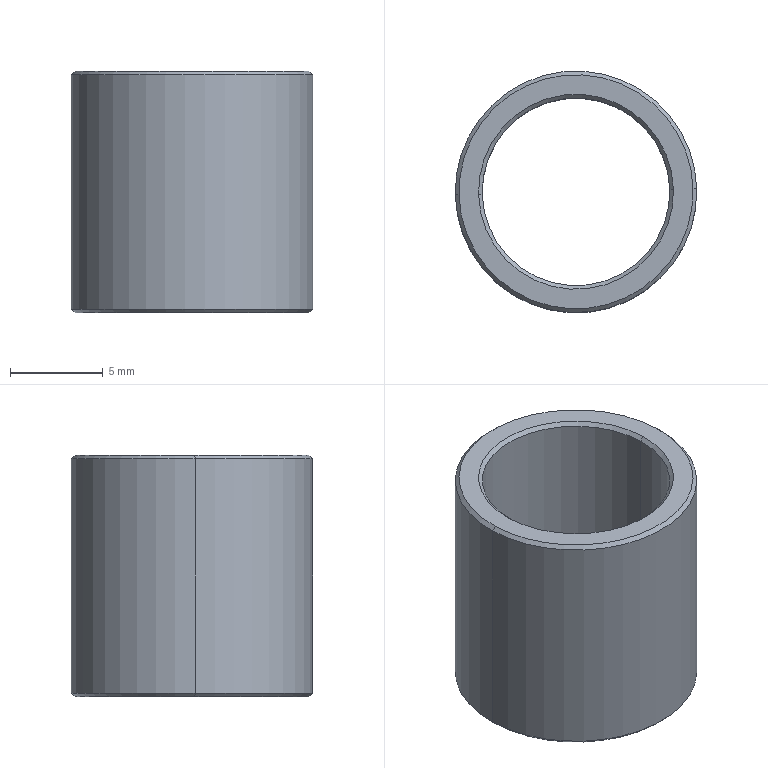Component | SolidWorks | 170423A4-IdlerAssembly5-10_170423A4-AxisCollar-1 | 1 solid | 14 faces | box 13 x 13 x 13 mm | volume 681 mm3 | cone 8 | cylinder 4 | plane 2 | commonest cylinder face diameters 10.1 x2 13 x2
build123d program:
from build123d import *

# Parameters (mm, degrees)
SKETCH1_R           = 6.5
SKETCH1_R_2         = 5.05
BOSS_EXTRUDE1_DEPTH = 13
CHAMFER1_SIZE       = 0.2


with BuildPart() as part:
    # Sketch1 → Boss-Extrude1 (new body)
    with BuildSketch(Plane.XY):
        with Locations(Location((0, 0, 0), (0, 0, 180))):
            Circle(SKETCH1_R)
        with Locations(Location((0, 0, 0), (0, 0, 180))):
            Circle(SKETCH1_R_2, mode=Mode.SUBTRACT)
    extrude(amount=BOSS_EXTRUDE1_DEPTH)

    # Chamfer1
    chamfer1_edges = [part.edges().sort_by_distance(p)[0] for p in [
        (6.5, 0, 0),
        (6.5, 0, 13),
        (5.05, 0, 0),
        (5.05, 0, 13),
    ]]
    chamfer(chamfer1_edges, length=CHAMFER1_SIZE)


solid = part.part

# Placed as in the assembly
solid = solid.moved(Location((-162.746, 8.712, 437.5), (0, 0, 0)))
STEP:
#1=COLOUR_RGB('',0.7922,0.8196,0.9333);
#2=FILL_AREA_STYLE_COLOUR('',#1);
#3=FILL_AREA_STYLE('',(#2));
#4=SURFACE_STYLE_FILL_AREA(#3);
#5=SURFACE_SIDE_STYLE('',(#4));
#6=SURFACE_STYLE_USAGE(.BOTH.,#5);
#7=PRESENTATION_STYLE_ASSIGNMENT((#6));
#8=CARTESIAN_POINT('',(-6.209,0.348,17.728));
#9=VERTEX_POINT('',#8);
#10=CARTESIAN_POINT('',(-6.606,0.3379,17.728));
#11=VERTEX_POINT('',#10);
#12=CARTESIAN_POINT('',(-6.407,0.343,17.728));
#13=DIRECTION('',(0.,0.,1.));
#14=DIRECTION('',(-0.9997,-0.02534,0.));
#15=AXIS2_PLACEMENT_3D('',#12,#13,#14);
#16=CIRCLE('',#15,0.1988);
#17=EDGE_CURVE('',#9,#11,#16,.T.);
#18=ORIENTED_EDGE('',*,*,#17,.F.);
#19=CARTESIAN_POINT('',(-6.201,0.3482,17.736));
#20=VERTEX_POINT('',#19);
#21=CARTESIAN_POINT('',(-6.209,0.348,17.728));
#22=DIRECTION('',(0.7069,0.01792,0.7071));
#23=VECTOR('',#22,39.37);
#24=LINE('',#21,#23);
#25=EDGE_CURVE('',#9,#20,#24,.T.);
#26=ORIENTED_EDGE('',*,*,#25,.T.);
#27=CARTESIAN_POINT('',(-6.614,0.3377,17.736));
#28=VERTEX_POINT('',#27);
#29=CARTESIAN_POINT('',(-6.407,0.343,17.736));
#30=DIRECTION('',(0.,0.,-1.));
#31=DIRECTION('',(-0.9997,-0.02534,0.));
#32=AXIS2_PLACEMENT_3D('',#29,#30,#31);
#33=CIRCLE('',#32,0.2067);
#34=EDGE_CURVE('',#28,#20,#33,.T.);
#35=ORIENTED_EDGE('',*,*,#34,.F.);
#36=CARTESIAN_POINT('',(-6.606,0.3379,17.728));
#37=DIRECTION('',(-0.7069,-0.01792,0.7071));
#38=VECTOR('',#37,39.37);
#39=LINE('',#36,#38);
#40=EDGE_CURVE('',#11,#28,#39,.T.);
#41=ORIENTED_EDGE('',*,*,#40,.F.);
#42=EDGE_LOOP('',(#18,#26,#35,#41));
#43=FACE_OUTER_BOUND('',#42,.T.);
#44=CARTESIAN_POINT('',(-6.407,0.343,17.728));
#45=DIRECTION('',(0.,0.,1.));
#46=DIRECTION('',(-0.9997,-0.02534,0.));
#47=AXIS2_PLACEMENT_3D('',#44,#45,#46);
#48=CONICAL_SURFACE('',#47,0.1988,0.7854);
#49=ADVANCED_FACE('',(#43),#48,.F.);
#50=CARTESIAN_POINT('',(-6.655,0.3367,17.736));
#51=VERTEX_POINT('',#50);
#52=CARTESIAN_POINT('',(-6.159,0.3493,17.736));
#53=VERTEX_POINT('',#52);
#54=CARTESIAN_POINT('',(-6.407,0.343,17.736));
#55=DIRECTION('',(0.,0.,1.));
#56=DIRECTION('',(-0.9997,-0.02534,0.));
#57=AXIS2_PLACEMENT_3D('',#54,#55,#56);
#58=CIRCLE('',#57,0.248);
#59=EDGE_CURVE('',#51,#53,#58,.T.);
#60=ORIENTED_EDGE('',*,*,#59,.F.);
#61=CARTESIAN_POINT('',(-6.663,0.3365,17.728));
#62=VERTEX_POINT('',#61);
#63=CARTESIAN_POINT('',(-6.655,0.3367,17.736));
#64=DIRECTION('',(-0.7069,-0.01792,-0.7071));
#65=VECTOR('',#64,39.37);
#66=LINE('',#63,#65);
#67=EDGE_CURVE('',#51,#62,#66,.T.);
#68=ORIENTED_EDGE('',*,*,#67,.T.);
#69=CARTESIAN_POINT('',(-6.152,0.3495,17.728));
#70=VERTEX_POINT('',#69);
#71=CARTESIAN_POINT('',(-6.407,0.343,17.728));
#72=DIRECTION('',(0.,0.,-1.));
#73=DIRECTION('',(-0.9997,-0.02534,0.));
#74=AXIS2_PLACEMENT_3D('',#71,#72,#73);
#75=CIRCLE('',#74,0.2559);
#76=EDGE_CURVE('',#70,#62,#75,.T.);
#77=ORIENTED_EDGE('',*,*,#76,.F.);
#78=CARTESIAN_POINT('',(-6.159,0.3493,17.736));
#79=DIRECTION('',(0.7069,0.01792,-0.7071));
#80=VECTOR('',#79,39.37);
#81=LINE('',#78,#80);
#82=EDGE_CURVE('',#53,#70,#81,.T.);
#83=ORIENTED_EDGE('',*,*,#82,.F.);
#84=EDGE_LOOP('',(#60,#68,#77,#83));
#85=FACE_OUTER_BOUND('',#84,.T.);
#86=CARTESIAN_POINT('',(-6.407,0.343,17.736));
#87=DIRECTION('',(0.,0.,-1.));
#88=DIRECTION('',(0.9997,0.02534,0.));
#89=AXIS2_PLACEMENT_3D('',#86,#87,#88);
#90=CONICAL_SURFACE('',#89,0.248,0.7854);
#91=ADVANCED_FACE('',(#85),#90,.T.);
#92=CARTESIAN_POINT('',(-6.159,0.3493,17.224));
#93=VERTEX_POINT('',#92);
#94=CARTESIAN_POINT('',(-6.655,0.3367,17.224));
#95=VERTEX_POINT('',#94);
#96=CARTESIAN_POINT('',(-6.407,0.343,17.224));
#97=DIRECTION('',(0.,0.,-1.));
#98=DIRECTION('',(-0.9997,-0.02534,0.));
#99=AXIS2_PLACEMENT_3D('',#96,#97,#98);
#100=CIRCLE('',#99,0.248);
#101=EDGE_CURVE('',#93,#95,#100,.T.);
#102=ORIENTED_EDGE('',*,*,#101,.F.);
#103=CARTESIAN_POINT('',(-6.152,0.3495,17.232));
#104=VERTEX_POINT('',#103);
#105=CARTESIAN_POINT('',(-6.152,0.3495,17.232));
#106=DIRECTION('',(0.7069,0.01792,0.7071));
#107=VECTOR('',#106,39.37);
#108=LINE('',#105,#107);
#109=EDGE_CURVE('',#93,#104,#108,.T.);
#110=ORIENTED_EDGE('',*,*,#109,.T.);
#111=CARTESIAN_POINT('',(-6.663,0.3365,17.232));
#112=VERTEX_POINT('',#111);
#113=CARTESIAN_POINT('',(-6.407,0.343,17.232));
#114=DIRECTION('',(0.,0.,1.));
#115=DIRECTION('',(-0.9997,-0.02534,0.));
#116=AXIS2_PLACEMENT_3D('',#113,#114,#115);
#117=CIRCLE('',#116,0.2559);
#118=EDGE_CURVE('',#112,#104,#117,.T.);
#119=ORIENTED_EDGE('',*,*,#118,.F.);
#120=CARTESIAN_POINT('',(-6.663,0.3365,17.232));
#121=DIRECTION('',(-0.7069,-0.01792,0.7071));
#122=VECTOR('',#121,39.37);
#123=LINE('',#120,#122);
#124=EDGE_CURVE('',#95,#112,#123,.T.);
#125=ORIENTED_EDGE('',*,*,#124,.F.);
#126=EDGE_LOOP('',(#102,#110,#119,#125));
#127=FACE_OUTER_BOUND('',#126,.T.);
#128=CARTESIAN_POINT('',(-6.407,0.343,17.232));
#129=DIRECTION('',(0.,0.,1.));
#130=DIRECTION('',(-0.9997,-0.02534,0.));
#131=AXIS2_PLACEMENT_3D('',#128,#129,#130);
#132=CONICAL_SURFACE('',#131,0.2559,0.7854);
#133=ADVANCED_FACE('',(#127),#132,.T.);
#134=CARTESIAN_POINT('',(-6.606,0.3379,17.232));
#135=VERTEX_POINT('',#134);
#136=CARTESIAN_POINT('',(-6.209,0.348,17.232));
#137=VERTEX_POINT('',#136);
#138=CARTESIAN_POINT('',(-6.407,0.343,17.232));
#139=DIRECTION('',(0.,0.,-1.));
#140=DIRECTION('',(-0.9997,-0.02534,0.));
#141=AXIS2_PLACEMENT_3D('',#138,#139,#140);
#142=CIRCLE('',#141,0.1988);
#143=EDGE_CURVE('',#135,#137,#142,.T.);
#144=ORIENTED_EDGE('',*,*,#143,.F.);
#145=CARTESIAN_POINT('',(-6.614,0.3377,17.224));
#146=VERTEX_POINT('',#145);
#147=CARTESIAN_POINT('',(-6.614,0.3377,17.224));
#148=DIRECTION('',(-0.7069,-0.01792,-0.7071));
#149=VECTOR('',#148,39.37);
#150=LINE('',#147,#149);
#151=EDGE_CURVE('',#135,#146,#150,.T.);
#152=ORIENTED_EDGE('',*,*,#151,.T.);
#153=CARTESIAN_POINT('',(-6.201,0.3482,17.224));
#154=VERTEX_POINT('',#153);
#155=CARTESIAN_POINT('',(-6.407,0.343,17.224));
#156=DIRECTION('',(0.,0.,1.));
#157=DIRECTION('',(-0.9997,-0.02534,0.));
#158=AXIS2_PLACEMENT_3D('',#155,#156,#157);
#159=CIRCLE('',#158,0.2067);
#160=EDGE_CURVE('',#154,#146,#159,.T.);
#161=ORIENTED_EDGE('',*,*,#160,.F.);
#162=CARTESIAN_POINT('',(-6.201,0.3482,17.224));
#163=DIRECTION('',(0.7069,0.01792,-0.7071));
#164=VECTOR('',#163,39.37);
#165=LINE('',#162,#164);
#166=EDGE_CURVE('',#137,#154,#165,.T.);
#167=ORIENTED_EDGE('',*,*,#166,.F.);
#168=EDGE_LOOP('',(#144,#152,#161,#167));
#169=FACE_OUTER_BOUND('',#168,.T.);
#170=CARTESIAN_POINT('',(-6.407,0.343,17.224));
#171=DIRECTION('',(0.,0.,-1.));
#172=DIRECTION('',(0.9997,0.02534,0.));
#173=AXIS2_PLACEMENT_3D('',#170,#171,#172);
#174=CONICAL_SURFACE('',#173,0.2067,0.7854);
#175=ADVANCED_FACE('',(#169),#174,.F.);
#176=ORIENTED_EDGE('',*,*,#17,.T.);
#177=CARTESIAN_POINT('',(-6.606,0.3379,17.736));
#178=DIRECTION('',(0.,0.,-1.));
#179=VECTOR('',#178,39.37);
#180=LINE('',#177,#179);
#181=EDGE_CURVE('',#11,#135,#180,.T.);
#182=ORIENTED_EDGE('',*,*,#181,.T.);
#183=ORIENTED_EDGE('',*,*,#143,.T.);
#184=CARTESIAN_POINT('',(-6.209,0.348,17.736));
#185=DIRECTION('',(0.,0.,-1.));
#186=VECTOR('',#185,39.37);
#187=LINE('',#184,#186);
#188=EDGE_CURVE('',#9,#137,#187,.T.);
#189=ORIENTED_EDGE('',*,*,#188,.F.);
#190=EDGE_LOOP('',(#176,#182,#183,#189));
#191=FACE_OUTER_BOUND('',#190,.T.);
#192=CARTESIAN_POINT('',(-6.407,0.343,17.736));
#193=DIRECTION('',(0.,0.,-1.));
#194=DIRECTION('',(0.9997,0.02534,0.));
#195=AXIS2_PLACEMENT_3D('',#192,#193,#194);
#196=CYLINDRICAL_SURFACE('',#195,0.1988);
#197=ADVANCED_FACE('',(#191),#196,.F.);
#198=ORIENTED_EDGE('',*,*,#76,.T.);
#199=CARTESIAN_POINT('',(-6.663,0.3365,17.736));
#200=DIRECTION('',(0.,0.,-1.));
#201=VECTOR('',#200,39.37);
#202=LINE('',#199,#201);
#203=EDGE_CURVE('',#62,#112,#202,.T.);
#204=ORIENTED_EDGE('',*,*,#203,.T.);
#205=ORIENTED_EDGE('',*,*,#118,.T.);
#206=CARTESIAN_POINT('',(-6.152,0.3495,17.736));
#207=DIRECTION('',(0.,0.,-1.));
#208=VECTOR('',#207,39.37);
#209=LINE('',#206,#208);
#210=EDGE_CURVE('',#70,#104,#209,.T.);
#211=ORIENTED_EDGE('',*,*,#210,.F.);
#212=EDGE_LOOP('',(#198,#204,#205,#211));
#213=FACE_OUTER_BOUND('',#212,.T.);
#214=CARTESIAN_POINT('',(-6.407,0.343,17.736));
#215=DIRECTION('',(0.,0.,-1.));
#216=DIRECTION('',(0.9997,0.02534,0.));
#217=AXIS2_PLACEMENT_3D('',#214,#215,#216);
#218=CYLINDRICAL_SURFACE('',#217,0.2559);
#219=ADVANCED_FACE('',(#213),#218,.T.);
#220=CARTESIAN_POINT('',(-6.407,0.343,17.736));
#221=DIRECTION('',(0.,0.,1.));
#222=DIRECTION('',(-0.9997,-0.02534,0.));
#223=AXIS2_PLACEMENT_3D('',#220,#221,#222);
#224=CIRCLE('',#223,0.248);
#225=EDGE_CURVE('',#53,#51,#224,.T.);
#226=ORIENTED_EDGE('',*,*,#225,.T.);
#227=ORIENTED_EDGE('',*,*,#59,.T.);
#228=EDGE_LOOP('',(#226,#227));
#229=FACE_OUTER_BOUND('',#228,.T.);
#230=ORIENTED_EDGE('',*,*,#34,.T.);
#231=CARTESIAN_POINT('',(-6.407,0.343,17.736));
#232=DIRECTION('',(0.,0.,-1.));
#233=DIRECTION('',(-0.9997,-0.02534,0.));
#234=AXIS2_PLACEMENT_3D('',#231,#232,#233);
#235=CIRCLE('',#234,0.2067);
#236=EDGE_CURVE('',#20,#28,#235,.T.);
#237=ORIENTED_EDGE('',*,*,#236,.T.);
#238=EDGE_LOOP('',(#230,#237));
#239=FACE_BOUND('',#238,.T.);
#240=CARTESIAN_POINT('',(-6.407,0.343,17.736));
#241=DIRECTION('',(0.,0.,1.));
#242=DIRECTION('',(-0.9997,-0.02534,0.));
#243=AXIS2_PLACEMENT_3D('',#240,#241,#242);
#244=PLANE('',#243);
#245=ADVANCED_FACE('',(#229,#239),#244,.T.);
#246=ORIENTED_EDGE('',*,*,#160,.T.);
#247=CARTESIAN_POINT('',(-6.407,0.343,17.224));
#248=DIRECTION('',(0.,0.,1.));
#249=DIRECTION('',(-0.9997,-0.02534,0.));
#250=AXIS2_PLACEMENT_3D('',#247,#248,#249);
#251=CIRCLE('',#250,0.2067);
#252=EDGE_CURVE('',#146,#154,#251,.T.);
#253=ORIENTED_EDGE('',*,*,#252,.T.);
#254=EDGE_LOOP('',(#246,#253));
#255=FACE_BOUND('',#254,.T.);
#256=CARTESIAN_POINT('',(-6.407,0.343,17.224));
#257=DIRECTION('',(0.,0.,-1.));
#258=DIRECTION('',(-0.9997,-0.02534,0.));
#259=AXIS2_PLACEMENT_3D('',#256,#257,#258);
#260=CIRCLE('',#259,0.248);
#261=EDGE_CURVE('',#95,#93,#260,.T.);
#262=ORIENTED_EDGE('',*,*,#261,.T.);
#263=ORIENTED_EDGE('',*,*,#101,.T.);
#264=EDGE_LOOP('',(#262,#263));
#265=FACE_OUTER_BOUND('',#264,.T.);
#266=CARTESIAN_POINT('',(-6.407,0.343,17.224));
#267=DIRECTION('',(0.,0.,1.));
#268=DIRECTION('',(-0.9997,-0.02534,0.));
#269=AXIS2_PLACEMENT_3D('',#266,#267,#268);
#270=PLANE('',#269);
#271=ADVANCED_FACE('',(#255,#265),#270,.F.);
#272=ORIENTED_EDGE('',*,*,#203,.F.);
#273=CARTESIAN_POINT('',(-6.407,0.343,17.728));
#274=DIRECTION('',(0.,0.,-1.));
#275=DIRECTION('',(-0.9997,-0.02534,0.));
#276=AXIS2_PLACEMENT_3D('',#273,#274,#275);
#277=CIRCLE('',#276,0.2559);
#278=EDGE_CURVE('',#62,#70,#277,.T.);
#279=ORIENTED_EDGE('',*,*,#278,.T.);
#280=ORIENTED_EDGE('',*,*,#210,.T.);
#281=CARTESIAN_POINT('',(-6.407,0.343,17.232));
#282=DIRECTION('',(0.,0.,1.));
#283=DIRECTION('',(-0.9997,-0.02534,0.));
#284=AXIS2_PLACEMENT_3D('',#281,#282,#283);
#285=CIRCLE('',#284,0.2559);
#286=EDGE_CURVE('',#104,#112,#285,.T.);
#287=ORIENTED_EDGE('',*,*,#286,.T.);
#288=EDGE_LOOP('',(#272,#279,#280,#287));
#289=FACE_OUTER_BOUND('',#288,.T.);
#290=CARTESIAN_POINT('',(-6.407,0.343,17.736));
#291=DIRECTION('',(0.,0.,-1.));
#292=DIRECTION('',(0.9997,0.02534,0.));
#293=AXIS2_PLACEMENT_3D('',#290,#291,#292);
#294=CYLINDRICAL_SURFACE('',#293,0.2559);
#295=ADVANCED_FACE('',(#289),#294,.T.);
#296=ORIENTED_EDGE('',*,*,#181,.F.);
#297=CARTESIAN_POINT('',(-6.407,0.343,17.728));
#298=DIRECTION('',(0.,0.,1.));
#299=DIRECTION('',(-0.9997,-0.02534,0.));
#300=AXIS2_PLACEMENT_3D('',#297,#298,#299);
#301=CIRCLE('',#300,0.1988);
#302=EDGE_CURVE('',#11,#9,#301,.T.);
#303=ORIENTED_EDGE('',*,*,#302,.T.);
#304=ORIENTED_EDGE('',*,*,#188,.T.);
#305=CARTESIAN_POINT('',(-6.407,0.343,17.232));
#306=DIRECTION('',(0.,0.,-1.));
#307=DIRECTION('',(-0.9997,-0.02534,0.));
#308=AXIS2_PLACEMENT_3D('',#305,#306,#307);
#309=CIRCLE('',#308,0.1988);
#310=EDGE_CURVE('',#137,#135,#309,.T.);
#311=ORIENTED_EDGE('',*,*,#310,.T.);
#312=EDGE_LOOP('',(#296,#303,#304,#311));
#313=FACE_OUTER_BOUND('',#312,.T.);
#314=CARTESIAN_POINT('',(-6.407,0.343,17.736));
#315=DIRECTION('',(0.,0.,-1.));
#316=DIRECTION('',(0.9997,0.02534,0.));
#317=AXIS2_PLACEMENT_3D('',#314,#315,#316);
#318=CYLINDRICAL_SURFACE('',#317,0.1988);
#319=ADVANCED_FACE('',(#313),#318,.F.);
#320=ORIENTED_EDGE('',*,*,#151,.F.);
#321=ORIENTED_EDGE('',*,*,#310,.F.);
#322=ORIENTED_EDGE('',*,*,#166,.T.);
#323=ORIENTED_EDGE('',*,*,#252,.F.);
#324=EDGE_LOOP('',(#320,#321,#322,#323));
#325=FACE_OUTER_BOUND('',#324,.T.);
#326=CARTESIAN_POINT('',(-6.407,0.343,17.224));
#327=DIRECTION('',(0.,0.,-1.));
#328=DIRECTION('',(0.9997,0.02534,0.));
#329=AXIS2_PLACEMENT_3D('',#326,#327,#328);
#330=CONICAL_SURFACE('',#329,0.2067,0.7854);
#331=ADVANCED_FACE('',(#325),#330,.F.);
#332=ORIENTED_EDGE('',*,*,#109,.F.);
#333=ORIENTED_EDGE('',*,*,#261,.F.);
#334=ORIENTED_EDGE('',*,*,#124,.T.);
#335=ORIENTED_EDGE('',*,*,#286,.F.);
#336=EDGE_LOOP('',(#332,#333,#334,#335));
#337=FACE_OUTER_BOUND('',#336,.T.);
#338=CARTESIAN_POINT('',(-6.407,0.343,17.232));
#339=DIRECTION('',(0.,0.,1.));
#340=DIRECTION('',(-0.9997,-0.02534,0.));
#341=AXIS2_PLACEMENT_3D('',#338,#339,#340);
#342=CONICAL_SURFACE('',#341,0.2559,0.7854);
#343=ADVANCED_FACE('',(#337),#342,.T.);
#344=ORIENTED_EDGE('',*,*,#67,.F.);
#345=ORIENTED_EDGE('',*,*,#225,.F.);
#346=ORIENTED_EDGE('',*,*,#82,.T.);
#347=ORIENTED_EDGE('',*,*,#278,.F.);
#348=EDGE_LOOP('',(#344,#345,#346,#347));
#349=FACE_OUTER_BOUND('',#348,.T.);
#350=CARTESIAN_POINT('',(-6.407,0.343,17.736));
#351=DIRECTION('',(0.,0.,-1.));
#352=DIRECTION('',(0.9997,0.02534,0.));
#353=AXIS2_PLACEMENT_3D('',#350,#351,#352);
#354=CONICAL_SURFACE('',#353,0.248,0.7854);
#355=ADVANCED_FACE('',(#349),#354,.T.);
#356=ORIENTED_EDGE('',*,*,#25,.F.);
#357=ORIENTED_EDGE('',*,*,#302,.F.);
#358=ORIENTED_EDGE('',*,*,#40,.T.);
#359=ORIENTED_EDGE('',*,*,#236,.F.);
#360=EDGE_LOOP('',(#356,#357,#358,#359));
#361=FACE_OUTER_BOUND('',#360,.T.);
#362=CARTESIAN_POINT('',(-6.407,0.343,17.728));
#363=DIRECTION('',(0.,0.,1.));
#364=DIRECTION('',(-0.9997,-0.02534,0.));
#365=AXIS2_PLACEMENT_3D('',#362,#363,#364);
#366=CONICAL_SURFACE('',#365,0.1988,0.7854);
#367=ADVANCED_FACE('',(#361),#366,.F.);
#368=CLOSED_SHELL('',(#49,#91,#133,#175,#197,#219,#245,#271,#295,#319,#331,#343,#355,#367));
#369=MANIFOLD_SOLID_BREP('',#368);
#370=STYLED_ITEM('',(#7),#369);
#371=(LENGTH_UNIT()NAMED_UNIT(*)SI_UNIT($,.METRE.));
#372=LENGTH_MEASURE_WITH_UNIT(LENGTH_MEASURE(0.0254),#371);
#373=DIMENSIONAL_EXPONENTS(1.,0.,0.,0.,0.,0.,0.);
#374=(CONVERSION_BASED_UNIT('',#372)LENGTH_UNIT()NAMED_UNIT(#373));
#375=UNCERTAINTY_MEASURE_WITH_UNIT(LENGTH_MEASURE(0.00001),#374,'','');
#376=(NAMED_UNIT(*)PLANE_ANGLE_UNIT()SI_UNIT($,.RADIAN.));
#377=(NAMED_UNIT(*)SI_UNIT($,.STERADIAN.)SOLID_ANGLE_UNIT());
#378=(GEOMETRIC_REPRESENTATION_CONTEXT(3)GLOBAL_UNCERTAINTY_ASSIGNED_CONTEXT((#375))GLOBAL_UNIT_ASSIGNED_CONTEXT((#374,#376,#377))REPRESENTATION_CONTEXT('',''));
#379=MECHANICAL_DESIGN_GEOMETRIC_PRESENTATION_REPRESENTATION('',(#370),#378);
#380=PRESENTATION_LAYER_ASSIGNMENT('','',(#370));
#381=CARTESIAN_POINT('',(0.,0.,0.));
#382=DIRECTION('',(0.,0.,1.));
#383=DIRECTION('',(1.,0.,0.));
#384=AXIS2_PLACEMENT_3D('',#381,#382,#383);
#385=(LENGTH_UNIT()NAMED_UNIT(*)SI_UNIT($,.METRE.));
#386=LENGTH_MEASURE_WITH_UNIT(LENGTH_MEASURE(0.0254),#385);
#387=DIMENSIONAL_EXPONENTS(1.,0.,0.,0.,0.,0.,0.);
#388=(CONVERSION_BASED_UNIT('',#386)LENGTH_UNIT()NAMED_UNIT(#387));
#389=UNCERTAINTY_MEASURE_WITH_UNIT(LENGTH_MEASURE(0.00001),#388,'','');
#390=(NAMED_UNIT(*)PLANE_ANGLE_UNIT()SI_UNIT($,.RADIAN.));
#391=(NAMED_UNIT(*)SI_UNIT($,.STERADIAN.)SOLID_ANGLE_UNIT());
#392=(GEOMETRIC_REPRESENTATION_CONTEXT(3)GLOBAL_UNCERTAINTY_ASSIGNED_CONTEXT((#389))GLOBAL_UNIT_ASSIGNED_CONTEXT((#388,#390,#391))REPRESENTATION_CONTEXT('',''));
#393=ADVANCED_BREP_SHAPE_REPRESENTATION('',(#369,#384),#392);